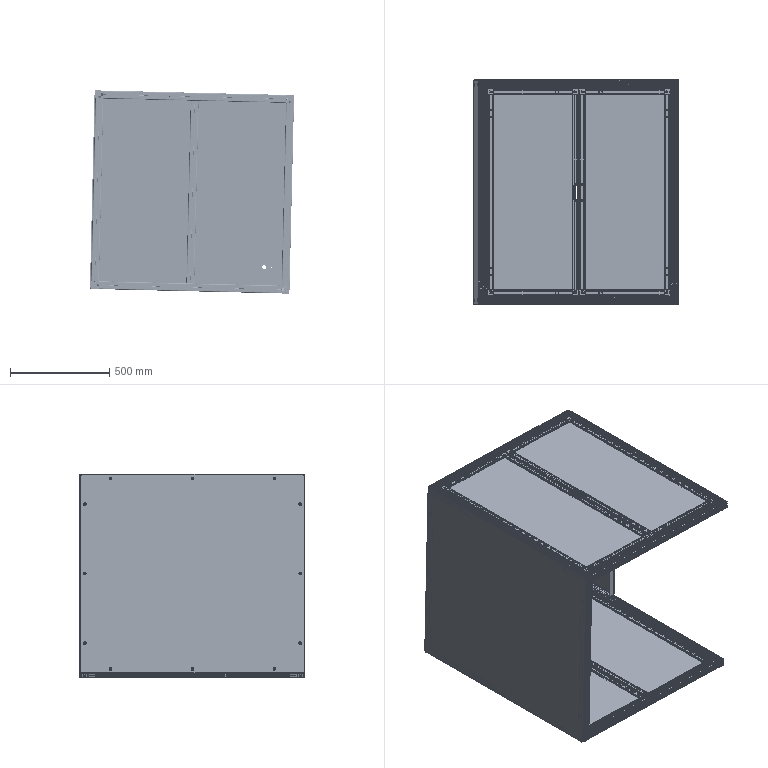Assembly | SolidWorks | mm | 149 component files | 149 solids | 6238 faces | box 1028.53 x 1130 x 1023.65 mm | volume 29494615 mm3 | plane 3910 | cylinder 1800 | cone 520 | spline 8 | commonest cylinder face diameters 6 x232 6.6 x230 2 x192 5 x184 11 x152 10 x120 6.8 x100 1 x96
Bill of materials:
1530ConnectorAMS12-1530 | 16 |  | Rectangular block with plain flat faces and round through-holes in its side faces.
ref18 | 4 | A6061 | Long, slender extruded bar with a rectangular cross-section and rounded corners. Each short side has an undercut slot pair, and there is a round bore through the center along its length. Small holes are grouped near both ends of one face.
AOB05-1530-L397 , Length 397mm | 2 | A6061 | Straight extruded bar with the same rounded-rectangle, two-slot cross-section and center bore as the slotted bars. No extra cutouts are visible along its length.
AOB05-1530-L397 , Length 397mm | 6 | A6061 | Straight extruded bar with a rounded-rectangle cross-section, undercut slots on two opposite sides and a central round bore. No extra cutouts are visible along its length.
1803ME3001 (Size:846*412*5mm) | 4 | PC | Thin flat rectangular plate with small step notches at each corner, so the short ends are slightly narrower.
AOB05-1530-L827-2 , Length 827mm | 4 | A6061 | Long extruded bar with the rounded-rectangle, two-slot cross-section and central bore. Mid-length, it has a rectangular cutout in one face with a small hole on each side of it.
HexSocketHeadCapScrewM6-16FerricOxide | 32 | SCM435 | Pin-shaped part with a short, larger-diameter cylindrical head and a smaller, longer cylindrical shank. Both ends are chamfered.
AOB05-4040-L920-LP-RP-LE-Z6-A70-B260-C260-D260 , Length 920mm | 1 | A6061 | Long extruded bar with a square cross-section, an undercut slot centered on each of the four sides, diagonal webs and a central bore with four radial notches. Small holes appear along one face and near the ends.
AOB05-4040-L920-LP-RP-LE-Z6-A70-B260-C260-D260 , Length 920mm | 2 | A6061 | Long extruded bar with a square cross-section, an undercut slot on each side, diagonal webs and a central notched bore. Small holes appear along one face and near the ends.
AOB05-4040-L970 , Length970mm | 4 | A6061 | Long straight extruded bar with a square cross-section, an undercut slot on each of the four sides, diagonal webs, hollow corner pockets and a central bore with four radial notches. No holes are visible along its length.
A3008 | 5 |  | Long straight extruded bar with a square cross-section, an undercut slot on each side, diagonal webs and a central notched bore. Small marks near the ends of one face may be holes.
Built-inConnectorADJ42-G408-D6.5 | 14 | S45C | Solid short cylinder with a round hole straight through its diameter. A thin rectangular tab sticks out sideways from the curved surface, flush with one end face.
HexSocketHeadCapScrewM6-25FerricOxide | 14 | SCM435 | Axisymmetric headed pin: short larger-diameter cylindrical head on a long, smooth, narrower cylindrical shank with a chamfered free end. Shaped like a cap-head screw blank.
RhombicNutAHG21-408-M6 | 14 |  | Rhombus/parallelogram-shaped block with one round through-hole near its center. The side profile is stepped, with a narrower raised tongue on one face. Two opposite corners of the outline are rounded and some edges are chamfered.
A3009 | 1 | PC | Thin, flat, nearly square plate with small rounded corners. It has a pattern of small holes spaced around the perimeter and one larger hole near a corner, surrounded by four small holes.
AHL21-308-M6 | 12 | S45C | Elongated half-round (D-section) body with a round through-hole crossing its curved side. A thin, angled flat flange extends from the top edge, and a small narrow rib or step runs along the flat back face. One edge has a semicircular notch where the hole breaks out.
HexSocketFlatHeadScrewM6-16FerrousOxide | 12 | SCM435 | Axisymmetric countersunk-head pin: a conical flat-topped head on a plain cylindrical shank with a chamfered tip. Shaped like a flat-head screw or rivet blank.
2403MA0512 | 1 | SUS304 | Tall rectangular bent-sheet panel with shallow depth, possibly a channel or tray shape with folded return flanges along its long sides. The main face has a rectangular cutout near the lower end, with a row of four round holes below it. The side flanges carry small round holes near the ends and the middle.
A3020 | 1 | PC | Thin, flat rectangular plate with small rounded corners and evenly spaced small holes around its perimeter, about three per edge. There are no interior features.
Mates:
1. coincident | assembly face at (597.759, -1214.138, 1384.919) dir (1, 0, 0) | assembly face at (597.759, -1307.138, 1248.419) dir (-1, 0, 0)
2. parallel | 2012MB0201-1/AUpperRackFrameModule-1/A3006-1 face at (-822.107, -81.15, -197.248) dir (0, -1, 0) | assembly plane at (0, 0, 0) dir (0, 1, 0)
3. coincident | 2012MB0201-1/AUpperRackFrameModule-1/A3007-2 face at (-1781.583, 1043.85, -163.887) dir (-0.9997, 0, 0.02392) | A3020-1 face at (-1793.436, 481.35, -659.245) dir (0.9997, 0, -0.02392)
4. coincident | 2012MB0201-1/AUpperRackFrameModule-1/A3007-2 face at (-1777.826, 1043.85, -194.986) dir (0, 1, 0) | A3020-1 face at (-1810.395, 1043.85, -1158.982) dir (0, 1, 0)
5. coincident | 2012MB0201-1/AUpperRackFrameModule-1/A3007-1 face at (-1800.898, 1043.85, -1159.21) dir (-0.02392, 0, -0.9997) | A3020-1 face at (-1810.395, 1043.85, -1158.982) dir (-0.02392, 0, -0.9997)
6. coincident | 2012MB0201-1/AUpperRackFrameModule-1/A3007-3 face at (-782.611, 1043.85, -218.799) dir (0.9997, 0, -0.02392) | 2403MA0512-1 face at (-793.722, 851.85, -683.166) dir (0.9997, 0, -0.02392)
7. coincident | 2012MB0201-1/AUpperRackFrameModule-1/A3008-3 face at (-787.217, 1003.85, -223.19) dir (0, -1, 0) | 2403MA0512-1 face at (-793.722, 1003.85, -683.166) dir (0, 1, 0)
8. distance | 2403MA0512-1 face at (-804.702, 851.85, -1142.035) dir (-0.02392, 0, -0.9997) | 2012MB0201-1/AUpperRackFrameModule-1/A3007-4 face at (-829.819, 1043.85, -1142.434) dir (0.02392, 0, 0.9997)
9. distance | ASideDoor-2-1/1530ConnectorAMS12-1530-8 face at (-482.615, 41.5, -1079.856) dir (0, -1, 0) | AUpperRackFrameModule-1/A3006-1 face at (-20.615, 40, -1084.356) dir (0, 1, 0)
10. distance | ASideDoor-2-1/1530ConnectorAMS12-1530-7 face at (-939.615, 41.5, -1094.856) dir (-1, 0, 0) | AUpperRackFrameModule-1/A3007-2 face at (-940.615, 1125, -1094.756) dir (1, 0, 0)
11. coincident | AUpperRackFrameModule-1/A3007-2 face at (-945.115, 1125, -1079.856) dir (0, 0, 1) | ASideDoor-2-1/A3001-4 face at (-939.615, 1053.5, -1079.856) dir (0, 0, 1)
12. distance | AUpperRackFrameModule-1/A3006-1 face at (-20.615, 40, -1084.356) dir (0, 1, 0) | ASideDoor-1-1/1530ConnectorAMS12-1530-8 face at (-21.615, 41.5, -1079.856) dir (0, -1, 0)
13. distance | ASideDoor-1-1/1530ConnectorAMS12-1530-8 face at (-21.615, 41.5, -1079.856) dir (1, 0, 0) | AUpperRackFrameModule-1/A3007-3 face at (-20.615, 1125, -1084.356) dir (-1, 0, 0)
14. coincident | AUpperRackFrameModule-1/A3007-3 face at (-5.715, 1125, -1079.856) dir (0, 0, 1) | ASideDoor-1-1/A3001-3 face at (-51.615, 1053.5, -1079.856) dir (0, 0, 1)
15. distance | UpperRackCoverModule-1/A3009-1 face at (-480.615, 1130, -1579.856) dir (0, 1, 0) | AUpperRackFrameModule-1/A3007-2 face at (-976.115, 1125, -1115.356) dir (0, 1, 0)
16. coincident | AUpperRackFrameModule-1/A3007-4 face at (-16.115, 1125, -2079.856) dir (0, 0, -1) | UpperRackCoverModule-1/A3009-1 face at (19.385, 1130, -2079.856) dir (0, 0, -1)
17. coincident | UpperRackCoverModule-1/A3009-1 face at (-980.615, 1130, -2079.856) dir (-1, 0, 0) | AUpperRackFrameModule-1/A3008-5 face at (-980.615, 1110.1, -1119.856) dir (-1, 0, 0)
18. parallel | AUpperRackFrameModule-1/A3008-6 face at (-20.615, 1120.5, -2063.956) dir (0, 0, 1) | UpperRackCoverModule-1/AHL21-308-M6-1 face at (-120.615, 1120.5, -2063.856) dir (0, 0, -1)
19. parallel | AUpperRackFrameModule-1/A3008-3 face at (3.485, 1120.5, -1119.856) dir (-1, 0, 0) | UpperRackCoverModule-1/AHL21-308-M6-2 face at (3.385, 1120.5, -1919.856) dir (1, 0, 0)
20. coincident | AUpperRackFrameModule-1/A3007-1 face at (-955.515, 1125, -2079.856) dir (0, 0, -1) | ASideDoor-1-3/A3001-3 face at (-909.115, 1053.5, -2079.856) dir (0, 0, -1)
21. coincident | ASideDoor-1-1/1530ConnectorAMS12-1530-5 face at (-478.615, 1083.5, -1079.856) dir (0, 1, 0) | ASideDoor-1-3/1530ConnectorAMS12-1530-5 face at (-482.115, 1083.5, -2079.856) dir (0, 1, 0)
22. coincident | AUpperRackFrameModule-1/A3007-4 face at (-16.115, 1125, -2079.856) dir (0, 0, -1) | ASideDoor-2-3/A3002-5 face at (-52.115, 1053.5, -2079.856) dir (0, 0, -1)
23. coincident | ASideDoor-2-3/1530ConnectorAMS12-1530-6 face at (-479.115, 1083.5, -2064.856) dir (0, 1, 0) | ASideDoor-1-3/1530ConnectorAMS12-1530-5 face at (-482.115, 1083.5, -2079.856) dir (0, 1, 0)
24. distance | ASideDoor-2-3/1530ConnectorAMS12-1530-5 face at (-22.115, 1083.5, -2079.856) dir (1, 0, 0) | AUpperRackFrameModule-1/A3007-4 face at (-20.615, 1125, -2064.956) dir (-1, 0, 0)
25. distance | ASideDoor-1-3/1530ConnectorAMS12-1530-6 face at (-939.115, 1083.5, -2064.856) dir (-1, 0, 0) | AUpperRackFrameModule-1/A3007-1 face at (-940.615, 1125, -2054.756) dir (1, 0, 0)
26. coincident | 2012MB0201 face at (-20.615, 0, -2075.356) dir (0, -1, 0) | 2012MB0201 plane at (0, 0, 0) dir (0, 1, 0)
27. coincident | A3005-1 face at (-200.853, 596.045, 717) dir (0, 1, 0) | 1530ConnectorAMS12-1530-5 face at (-215.853, 596.045, 724.5) dir (0, -1, 0)
28. coincident | A3005-1 face at (-215.853, 596.045, 724.5) dir (0, 0, 1) | 1530ConnectorAMS12-1530-5 face at (-200.853, 611.045, 724.5) dir (0, 0, 1)
29. coincident | A3005-1 face at (-215.853, 596.045, 709.5) dir (-1, 0, 0) | 1530ConnectorAMS12-1530-5 face at (-215.853, 626.045, 724.5) dir (-1, 0, 0)
30. coincident | A3001-3 face at (211.147, 596.045, 724.5) dir (0, 0, 1) | 1530ConnectorAMS12-1530-6 face at (226.147, 611.045, 724.5) dir (0, 0, 1)
31. coincident | A3001-3 face at (226.147, 596.045, 717) dir (0, 1, 0) | 1530ConnectorAMS12-1530-6 face at (241.147, 596.045, 709.5) dir (0, -1, 0)
32. coincident | A3001-3 face at (241.147, 596.045, 709.5) dir (1, 0, 0) | 1530ConnectorAMS12-1530-6 face at (241.147, 626.045, 709.5) dir (1, 0, 0)
33. coincident | A3005-1 face at (-200.853, -385.955, 717) dir (0, -1, 0) | 1530ConnectorAMS12-1530-7 face at (-215.853, -385.955, 709.5) dir (0, 1, 0)
34. coincident | A3001-3 face at (226.147, -385.955, 717) dir (0, -1, 0) | 1530ConnectorAMS12-1530-8 face at (241.147, -385.955, 724.5) dir (0, 1, 0)
35. distance | ASideDoor-1 face at (-61.253, -57.855, 719.5) dir (0, 0, 1) | A3005-1 face at (-185.853, 596.045, 720.25) dir (0, 0, -1)
36. distance | A3005-1 face at (-194.253, 596.045, 711.7) dir (1, 0, 0) | ASideDoor-1 face at (-194.253, 278.645, 719.5) dir (-1, 0, 0)
37. concentric | A3005-1 face at (-200.853, 69.545, 724.5) dir (0, 0, 1) r 2.5 | ASideDoor-1 face at (-200.853, 69.545, 724.5) dir (0, 0, 1) r 1.621
38. coincident | A3005-1 face at (-215.853, 596.045, 724.5) dir (0, 0, 1) | ASideDoor-1 face at (-196.353, 69.545, 724.5) dir (0, 0, -1)
39. parallel | 1530ConnectorAMS12-1530-8 face at (241.147, -415.955, 724.5) dir (0, -1, 0) | A3002-7 face at (211.147, -385.955, 709.5) dir (0, 1, 0)
40. coincident | A3005-1 face at (-215.853, 596.045, 709.5) dir (-1, 0, 0) | 1530ConnectorAMS12-1530-7 face at (-215.853, -415.955, 709.5) dir (-1, 0, 0)
41. coincident | A3001-3 face at (241.147, 596.045, 709.5) dir (1, 0, 0) | 1530ConnectorAMS12-1530-8 face at (241.147, -415.955, 724.5) dir (1, 0, 0)
42. coincident | A3005-1 face at (-215.853, 596.045, 709.5) dir (0, 0, -1) | 1530ConnectorAMS12-1530-7 face at (-200.853, -400.955, 709.5) dir (0, 0, -1)
43. coincident | A3005-1 face at (-215.853, 596.045, 724.5) dir (0, 0, 1) | A3002-7 face at (211.147, -385.955, 724.5) dir (0, 0, 1)
44. parallel | 1530ConnectorAMS12-1530-7 face at (-215.853, -415.955, 709.5) dir (0, -1, 0) | A3002-7 face at (211.147, -415.955, 709.5) dir (0, -1, 0)
45. coincident | A3005-1 face at (-185.853, 596.045, 709.5) dir (1, 0, 0) | A3002-7 face at (-185.853, -400.955, 717) dir (-1, 0, 0)
46. coincident | 1530ConnectorAMS12-1530-7 face at (-215.853, -415.955, 709.5) dir (0, -1, 0) | A3002-7 face at (211.147, -415.955, 709.5) dir (0, -1, 0)
47. coincident | A3001-3 face at (211.147, 596.045, 709.5) dir (0, 0, -1) | 1530ConnectorAMS12-1530-8 face at (226.147, -400.955, 709.5) dir (0, 0, -1)
48. coincident | 1530ConnectorAMS12-1530-6 face at (215.147, 611.045, 713.7) dir (1, 0, 0) | HexSocketHeadCapScrewM6-16FerricOxide-4 face at (215.147, 610.097, 712.091) dir (-1, 0, 0)
49. concentric | 1530ConnectorAMS12-1530-6 face at (226.147, 626.045, 717) dir (0, 1, 0) r 5.5 | HexSocketHeadCapScrewM6-16FerricOxide-3 face at (226.147, 600.045, 717) dir (0, 1, 0) r 5
50. coincident | 1530ConnectorAMS12-1530-6 face at (222.847, 600.045, 717) dir (0, 1, 0) | HexSocketHeadCapScrewM6-16FerricOxide-3 face at (226.867, 600.045, 712.052) dir (0, -1, 0)
51. coincident | 1530ConnectorAMS12-1530-5 face at (-189.853, 611.045, 720.3) dir (-1, 0, 0) | HexSocketHeadCapScrewM6-16FerricOxide-1 face at (-189.853, 613.137, 712.459) dir (1, 0, 0)
52. concentric | 1530ConnectorAMS12-1530-5 face at (-200.853, 626.045, 717) dir (0, 1, 0) r 5.5 | HexSocketHeadCapScrewM6-16FerricOxide-2 face at (-200.853, 500.045, 717) dir (0, 1, 0) r 3
53. coincident | 1530ConnectorAMS12-1530-5 face at (-197.553, 600.045, 717) dir (0, 1, 0) | HexSocketHeadCapScrewM6-16FerricOxide-2 face at (-205.814, 600.045, 716.38) dir (0, -1, 0)
54. concentric | 1530ConnectorAMS12-1530-7 face at (-200.853, -415.955, 717) dir (0, -1, 0) r 5.5 | HexSocketHeadCapScrewM6-16FerricOxide-5 face at (-200.853, -289.955, 717) dir (0, -1, 0) r 3
55. concentric | 1530ConnectorAMS12-1530-7 face at (-215.853, -400.955, 717) dir (-1, 0, 0) r 5.5 | HexSocketHeadCapScrewM6-16FerricOxide-6 face at (-89.853, -400.955, 717) dir (-1, 0, 0) r 3
56. coincident | 1530ConnectorAMS12-1530-7 face at (-189.853, -400.955, 713.7) dir (-1, 0, 0) | HexSocketHeadCapScrewM6-16FerricOxide-6 face at (-189.853, -400.955, 712) dir (1, 0, 0)
57. coincident | 1530ConnectorAMS12-1530-7 face at (-197.553, -389.955, 717) dir (0, -1, 0) | HexSocketHeadCapScrewM6-16FerricOxide-5 face at (-198.118, -389.955, 712.814) dir (0, 1, 0)
58. concentric | 1530ConnectorAMS12-1530-8 face at (241.147, -400.955, 717) dir (1, 0, 0) r 5.5 | HexSocketHeadCapScrewM6-16FerricOxide-7 face at (115.147, -400.955, 717) dir (1, 0, 0) r 3
59. coincident | 1530ConnectorAMS12-1530-8 face at (215.147, -400.955, 720.3) dir (1, 0, 0) | HexSocketHeadCapScrewM6-16FerricOxide-7 face at (215.147, -398.852, 712.464) dir (-1, 0, 0)
60. concentric | A3001-3 face at (226.147, 596.045, 717) dir (0, -1, 0) r 2.5 | HexSocketHeadCapScrewM6-16FerricOxide-8 face at (226.147, -289.955, 717) dir (0, -1, 0) r 3
61. coincident | 1530ConnectorAMS12-1530-8 face at (222.847, -389.955, 717) dir (0, -1, 0) | HexSocketHeadCapScrewM6-16FerricOxide-8 face at (229.723, -389.955, 720.495) dir (0, 1, 0)
62. coincident | 1530ConnectorAMS12-1530-5 face at (-185.853, 626.045, 724.5) dir (1, 0, 0) | A3002-0-1 face at (-185.853, 611.045, 717) dir (-1, 0, 0)
63. concentric | HexSocketHeadCapScrewM6-16FerricOxide-1 face at (-89.853, 611.045, 717) dir (-1, 0, 0) r 3 | A3002-0-1 face at (211.147, 611.045, 717) dir (-1, 0, 0) r 2.5
64. coincident | 1530ConnectorAMS12-1530-5 face at (-215.853, 626.045, 724.5) dir (0, 1, 0) | A3002-0-1 face at (211.147, 626.045, 709.5) dir (0, 1, 0)
65. coincident | 1530ConnectorAMS12-1530-6 face at (211.147, 626.045, 709.5) dir (-1, 0, 0) | A3002-0-1 face at (211.147, 611.045, 717) dir (1, 0, 0)
66. coincident | 1530ConnectorAMS12-1530-6 face at (241.147, 626.045, 709.5) dir (0, 1, 0) | A3002-0-1 face at (211.147, 626.045, 709.5) dir (0, 1, 0)
67. coincident | A3001-3 face at (211.147, 596.045, 724.5) dir (0, 0, 1) | A3002-0-1 face at (211.147, 626.045, 724.5) dir (0, 0, 1)
68. coincident | A3005-1 face at (-215.853, 596.045, 724.5) dir (0, 0, 1) | A3002-0-1 face at (211.147, 626.045, 724.5) dir (0, 0, 1)
69. coincident | A3001-4 face at (-200.853, 596.045, 717) dir (0, 1, 0) | 1530ConnectorAMS12-1530-5 face at (-215.853, 596.045, 724.5) dir (0, -1, 0)
70. coincident | A3001-4 face at (-215.853, 596.045, 724.5) dir (0, 0, 1) | 1530ConnectorAMS12-1530-5 face at (-200.853, 611.045, 724.5) dir (0, 0, 1)
71. coincident | A3001-4 face at (-215.853, 596.045, 709.5) dir (-1, 0, 0) | 1530ConnectorAMS12-1530-5 face at (-215.853, 626.045, 724.5) dir (-1, 0, 0)
72. coincident | A3002-5 face at (-185.853, 611.045, 717) dir (-1, 0, 0) | 1530ConnectorAMS12-1530-5 face at (-185.853, 626.045, 724.5) dir (1, 0, 0)
73. coincident | A3002-5 face at (-185.853, 596.045, 724.5) dir (0, 0, 1) | 1530ConnectorAMS12-1530-5 face at (-200.853, 611.045, 724.5) dir (0, 0, 1)
74. coincident | A3002-5 face at (-185.853, 626.045, 709.5) dir (0, 1, 0) | 1530ConnectorAMS12-1530-5 face at (-215.853, 626.045, 724.5) dir (0, 1, 0)
75. coincident | A3002-5 face at (211.147, 611.045, 717) dir (1, 0, 0) | 1530ConnectorAMS12-1530-6 face at (211.147, 626.045, 709.5) dir (-1, 0, 0)
76. coincident | A3002-5 face at (-185.853, 596.045, 724.5) dir (0, 0, 1) | 1530ConnectorAMS12-1530-6 face at (226.147, 611.045, 724.5) dir (0, 0, 1)
77. coincident | A3002-5 face at (-185.853, 626.045, 709.5) dir (0, 1, 0) | 1530ConnectorAMS12-1530-6 face at (241.147, 626.045, 709.5) dir (0, 1, 0)
78. coincident | A3005-2 face at (211.147, 596.045, 724.5) dir (0, 0, 1) | 1530ConnectorAMS12-1530-6 face at (226.147, 611.045, 724.5) dir (0, 0, 1)
79. coincident | A3005-2 face at (226.147, 596.045, 717) dir (0, 1, 0) | 1530ConnectorAMS12-1530-6 face at (241.147, 596.045, 709.5) dir (0, -1, 0)
80. coincident | A3005-2 face at (241.147, 596.045, 709.5) dir (1, 0, 0) | 1530ConnectorAMS12-1530-6 face at (241.147, 626.045, 709.5) dir (1, 0, 0)
81. coincident | A3001-4 face at (-215.853, 596.045, 724.5) dir (0, 0, 1) | A3002-6 face at (-185.853, -415.955, 724.5) dir (0, 0, 1)
82. coincident | A3001-4 face at (-185.853, 596.045, 709.5) dir (1, 0, 0) | A3002-6 face at (-185.853, -400.955, 717) dir (-1, 0, 0)
83. coincident | A3001-4 face at (-200.853, -385.955, 717) dir (0, -1, 0) | A3002-6 face at (-185.853, -385.955, 709.5) dir (0, 1, 0)
84. coincident | A3001-4 face at (-200.853, -385.955, 717) dir (0, -1, 0) | 1530ConnectorAMS12-1530-7 face at (-215.853, -385.955, 709.5) dir (0, 1, 0)
85. coincident | 1530ConnectorAMS12-1530-7 face at (-185.853, -415.955, 709.5) dir (1, 0, 0) | A3002-6 face at (-185.853, -400.955, 717) dir (-1, 0, 0)
86. coincident | 1530ConnectorAMS12-1530-7 face at (-200.853, -400.955, 724.5) dir (0, 0, 1) | A3002-6 face at (-185.853, -415.955, 724.5) dir (0, 0, 1)
87. coincident | A3005-2 face at (226.147, -385.955, 717) dir (0, -1, 0) | 1530ConnectorAMS12-1530-8 face at (241.147, -385.955, 724.5) dir (0, 1, 0)
88. coincident | 1530ConnectorAMS12-1530-8 face at (211.147, -415.955, 724.5) dir (-1, 0, 0) | A3002-6 face at (211.147, -400.955, 717) dir (1, 0, 0)
89. coincident | 1530ConnectorAMS12-1530-8 face at (226.147, -400.955, 724.5) dir (0, 0, 1) | A3002-6 face at (-185.853, -415.955, 724.5) dir (0, 0, 1)
90. width | A3002-6 face at (-185.853, -396.755, 714.074) dir (0, 1, 0) | A3002-5 face at (-185.853, 606.845, 714.074) dir (0, -1, 0) | A3004-2 face at (-193.353, -395.455, 719.5) dir (0, -1, 0) | A3004-2 face at (-193.353, 605.545, 719.5) dir (0, 1, 0)
91. width | A3001-4 face at (-196.653, 596.045, 714.074) dir (1, 0, 0) | A3005-2 face at (221.947, 596.045, 714.074) dir (-1, 0, 0) | A3004-2 face at (-193.353, 605.545, 719.5) dir (-1, 0, 0) | A3004-2 face at (218.647, 605.545, 719.5) dir (1, 0, 0)
92. width | A3005-2 face at (211.147, 596.045, 720.25) dir (0, 0, -1) | A3005-2 face at (211.147, 596.045, 713.75) dir (0, 0, 1) | A3004-2 face at (12.647, 105.045, 719.5) dir (0, 0, 1) | A3004-2 face at (12.647, 105.045, 714.5) dir (0, 0, -1)
93. concentric | 1530ConnectorAMS12-1530-8 face at (241.147, -400.955, 717) dir (1, 0, 0) r 5.5 | HexSocketHeadCapScrewM6-16FerricOxide-22 face at (215.147, -400.955, 717) dir (1, 0, 0) r 5
94. concentric | 1530ConnectorAMS12-1530-8 face at (226.147, -415.955, 717) dir (0, -1, 0) r 5.5 | HexSocketHeadCapScrewM6-16FerricOxide-23 face at (226.147, -389.955, 717) dir (0, -1, 0) r 5
95. coincident | 1530ConnectorAMS12-1530-8 face at (215.147, -400.955, 720.3) dir (1, 0, 0) | HexSocketHeadCapScrewM6-16FerricOxide-22 face at (215.147, -404.001, 720.965) dir (-1, 0, 0)
96. coincident | 1530ConnectorAMS12-1530-8 face at (222.847, -389.955, 717) dir (0, -1, 0) | HexSocketHeadCapScrewM6-16FerricOxide-23 face at (221.944, -389.955, 719.708) dir (0, 1, 0)
97. concentric | 1530ConnectorAMS12-1530-5 face at (-200.853, 626.045, 717) dir (0, 1, 0) r 5.5 | HexSocketHeadCapScrewM6-16FerricOxide-19 face at (-200.853, 500.045, 717) dir (0, 1, 0) r 3
98. coincident | 1530ConnectorAMS12-1530-5 face at (-197.553, 600.045, 717) dir (0, 1, 0) | HexSocketHeadCapScrewM6-16FerricOxide-19 face at (-204.91, 600.045, 719.922) dir (0, -1, 0)
99. concentric | 1530ConnectorAMS12-1530-7 face at (-215.853, -400.955, 717) dir (-1, 0, 0) r 5.5 | HexSocketHeadCapScrewM6-16FerricOxide-24 face at (-89.853, -400.955, 717) dir (-1, 0, 0) r 3
100. concentric | 1530ConnectorAMS12-1530-7 face at (-200.853, -415.955, 717) dir (0, -1, 0) r 5.5 | HexSocketHeadCapScrewM6-16FerricOxide-25 face at (-200.853, -289.955, 717) dir (0, -1, 0) r 3
101. coincident | 1530ConnectorAMS12-1530-7 face at (-197.553, -389.955, 717) dir (0, -1, 0) | HexSocketHeadCapScrewM6-16FerricOxide-25 face at (-205.36, -389.955, 719.164) dir (0, 1, 0)
102. coincident | 1530ConnectorAMS12-1530-7 face at (-189.853, -400.955, 713.7) dir (-1, 0, 0) | HexSocketHeadCapScrewM6-16FerricOxide-24 face at (-189.853, -398.844, 712.467) dir (1, 0, 0)
103. concentric | 1530ConnectorAMS12-1530-6 face at (241.147, 611.045, 717) dir (1, 0, 0) r 5.5 | HexSocketHeadCapScrewM6-16FerricOxide-21 face at (215.147, 611.045, 717) dir (1, 0, 0) r 5
104. coincident | 1530ConnectorAMS12-1530-6 face at (215.147, 611.045, 713.7) dir (1, 0, 0) | HexSocketHeadCapScrewM6-16FerricOxide-21 face at (215.147, 613.954, 721.067) dir (-1, 0, 0)
105. concentric | 1530ConnectorAMS12-1530-6 face at (226.147, 626.045, 717) dir (0, 1, 0) r 5.5 | HexSocketHeadCapScrewM6-16FerricOxide-20 face at (226.147, 600.045, 717) dir (0, 1, 0) r 5
106. coincident | 1530ConnectorAMS12-1530-6 face at (222.847, 600.045, 717) dir (0, 1, 0) | HexSocketHeadCapScrewM6-16FerricOxide-20 face at (231.141, 600.045, 716.755) dir (0, -1, 0)
107. concentric | 1530ConnectorAMS12-1530-5 face at (-215.853, 611.045, 717) dir (-1, 0, 0) r 5.5 | HexSocketHeadCapScrewM6-16FerricOxide-18 face at (-189.853, 611.045, 717) dir (-1, 0, 0) r 5
108. coincident | 1530ConnectorAMS12-1530-5 face at (-189.853, 611.045, 720.3) dir (-1, 0, 0) | HexSocketHeadCapScrewM6-16FerricOxide-18 face at (-189.853, 608.692, 721.412) dir (1, 0, 0)
109. coincident | A3006-1 face at (1026.374, 4.5, -29.823) dir (1, 0, 0) | A3007-2 face at (1026.374, 1125, -50.423) dir (-1, 0, 0)
110. coincident | A3006-1 face at (106.374, 25.1, -65.323) dir (0, 0, -1) | A3007-2 face at (1030.874, 1125, -65.323) dir (0, 0, -1)
111. coincident | A3006-1 face at (106.374, 4.5, -65.323) dir (0, 0, -1) | A3007-3 face at (91.474, 1125, -65.323) dir (0, 0, -1)
112. coincident | A3006-1 face at (106.374, 4.5, -29.823) dir (-1, 0, 0) | A3007-3 face at (106.374, 1125, -60.823) dir (1, 0, 0)
113. coincident | A3006-1 face at (106.374, 0, -50.423) dir (0, -1, 0) | A3007-2 face at (1061.874, 0, -29.823) dir (0, -1, 0)
114. coincident | A3006-1 face at (106.374, 4.5, -29.823) dir (-1, 0, 0) | A3007-3 face at (106.374, 1125, -60.823) dir (1, 0, 0)
115. coincident | A3006-1 face at (106.374, 0, -50.423) dir (0, -1, 0) | A3007-3 face at (101.874, 0, -29.823) dir (0, -1, 0)
116. coincident | A3006-1 face at (106.374, 40, -60.823) dir (0, 1, 0) | ADJ42-G408-D6.5Assembly-4/Built-inConnectorADJ42-G408-D6.5-1 face at (125.374, 40, -36.072) dir (0, 1, 0)
117. coincident | A3006-1 face at (106.374, 40, -40.223) dir (0, 1, 0) | ADJ42-G408-D6.5Assembly-5/Built-inConnectorADJ42-G408-D6.5-1 face at (1007.374, 40, -54.572) dir (0, 1, 0)
118. coincident | A3007-1 face at (1061.874, 1125, 934.677) dir (0, 0, 1) | A3008-6 face at (106.374, 1120.5, 934.677) dir (0, 0, 1)
119. coincident | A3007-1 face at (1026.374, 1125, 930.177) dir (-1, 0, 0) | A3008-6 face at (1026.374, 1089.5, 930.177) dir (1, 0, 0)
120. coincident | A3007-2 face at (1061.874, 1125, -29.823) dir (0, 1, 0) | A3008-5 face at (1041.274, 1125, -25.323) dir (0, 1, 0)
121. coincident | A3007-2 face at (1066.374, 1125, -60.823) dir (1, 0, 0) | A3008-5 face at (1066.374, 1110.1, -25.323) dir (1, 0, 0)
122. coincident | A3007-2 face at (1061.874, 1125, -25.323) dir (0, 0, 1) | A3008-5 face at (1030.874, 1089.5, -25.323) dir (0, 0, -1)
123. coincident | A3007-2 face at (1061.874, 1125, -29.823) dir (0, 1, 0) | A3008-7 face at (106.374, 1125, -40.223) dir (0, 1, 0)
124. coincident | A3007-2 face at (1051.474, 1125, -65.323) dir (0, 0, -1) | A3008-7 face at (106.374, 1110.1, -65.323) dir (0, 0, -1)
125. coincident | A3007-2 face at (1026.374, 1125, -50.423) dir (-1, 0, 0) | A3008-7 face at (1026.374, 1089.5, -29.823) dir (1, 0, 0)
126. coincident | A3007-2 face at (1030.874, 1125, -51.923) dir (1, 0, 0) | AUpperRackFrameModule face at (1031.124, 1125, -55.073) dir (-1, 0, 0)
127. width | AUpperRackFrameModule face at (1028.124, 1125, -41.323) dir (0, 0, 1) | AUpperRackFrameModule face at (1031.124, 1125, -49.323) dir (0, 0, -1) | A3007-2 face at (1030.874, 1125, -49.423) dir (0, 0, 1) | A3007-2 face at (1027.374, 1125, -41.223) dir (0, 0, -1)
128. coincident | A3007-2 edge at (1030.874, 1125, -41.223) dir (0, -1, 0) | AUpperRackFrameModule face at (1031.124, 42, -41.072) dir (-1, 0, 0)
129. coincident | A3007-2 face at (1061.874, 1125, -29.823) dir (0, 1, 0) | AUpperRackFrameModule face at (1037.624, 1125, -35.573) dir (0, 1, 0)
130. coincident | A3007-3 face at (101.874, 1125, -29.823) dir (0, 1, 0) | A3008-3 face at (101.874, 1125, -25.323) dir (0, 1, 0)
131. coincident | A3007-3 face at (66.374, 1125, -50.423) dir (-1, 0, 0) | A3008-3 face at (66.374, 1120.5, -25.323) dir (-1, 0, 0)
132. coincident | A3007-3 face at (101.874, 1125, -25.323) dir (0, 0, 1) | A3008-3 face at (70.874, 1089.5, -25.323) dir (0, 0, -1)
133. coincident | A3007-3 face at (101.874, 1125, -49.423) dir (-1, 0, 0) | AUpperRackFrameModule face at (102.124, 1125, -49.572) dir (1, 0, 0)
134. width | A3007-3 face at (90.474, 1125, -26.323) dir (-1, 0, 0) | A3007-3 face at (82.274, 1125, -29.823) dir (1, 0, 0) | AUpperRackFrameModule face at (82.624, 1125, -29.823) dir (-1, 0, 0) | AUpperRackFrameModule face at (90.624, 1125, -26.823) dir (1, 0, 0)
135. coincident | A3007-3 face at (90.474, 1125, -29.823) dir (0, 0, -1) | AUpperRackFrameModule face at (90.624, 1125, -29.823) dir (0, 0, 1)
136. coincident | A3007-3 face at (101.874, 1125, -29.823) dir (0, 1, 0) | AUpperRackFrameModule face at (95.624, 1125, -55.322) dir (0, 1, 0)
137. coincident | A3007-3 edge at (101.874, 1125, -41.223) dir (0, -1, 0) | AUpperRackFrameModule face at (106.729, 42, -28.427) dir (0.9409, 0, -0.3386)
138. coincident | A3007-3 face at (101.874, 1125, -29.823) dir (0, 1, 0) | AUpperRackFrameModule face at (96.374, 1125, -36.323) dir (0, 1, 0)
139. coincident | A3007-4 face at (101.874, 1125, 930.177) dir (0, 1, 0) | A3008-6 face at (106.374, 1125, 899.177) dir (0, 1, 0)
140. coincident | A3007-4 face at (70.874, 1125, 894.677) dir (0, 0, -1) | A3008-3 face at (70.874, 1089.5, 894.677) dir (0, 0, 1)
141. coincident | A3007-4 face at (106.374, 1125, 919.777) dir (1, 0, 0) | A3008-6 face at (106.374, 1089.5, 930.177) dir (-1, 0, 0)
142. coincident | A3007-4 face at (101.874, 1125, 934.677) dir (0, 0, 1) | A3008-6 face at (106.374, 1120.5, 934.677) dir (0, 0, 1)
143. width | A3007-4 face at (82.274, 1125, 895.677) dir (1, 0, 0) | A3007-4 face at (90.474, 1125, 899.177) dir (-1, 0, 0) | AUpperRackFrameModule face at (82.374, 1125, 896.177) dir (-1, 0, 0) | AUpperRackFrameModule face at (90.374, 1125, 899.177) dir (1, 0, 0)
144. coincident | A3007-4 face at (82.274, 1125, 899.177) dir (0, 0, 1) | AUpperRackFrameModule face at (82.374, 1125, 899.177) dir (0, 0, -1)
145. coincident | A3007-4 face at (101.874, 1125, 930.177) dir (0, 1, 0) | AUpperRackFrameModule face at (76.624, 1125, 905.677) dir (0, 1, 0)
146. concentric | A3008-7 face at (125.374, 1107, -45.322) dir (0, 1, 0) r 9.5 | ADJ42-G408-D6.5Assembly-1/Built-inConnectorADJ42-G408-D6.5-1 face at (125.374, 1123, -45.322) dir (0, -1, 0) r 9.25
147. coincident | A3008-7 face at (106.374, 1125, -40.223) dir (0, 1, 0) | A3008-8 face at (581.874, 1125, -25.323) dir (0, 1, 0)
148. coincident | A3008-7 face at (106.374, 1120.5, -25.323) dir (0, 0, 1) | A3008-8 face at (550.874, 1120.5, -25.323) dir (0, 0, -1)
149. concentric | A3008-5 face at (1046.373, 1107, -6.323) dir (0, 1, 0) r 9.5 | ADJ42-G408-D6.5Assembly-12/Built-inConnectorADJ42-G408-D6.5-1 face at (1046.373, 1123, -6.323) dir (0, -1, 0) r 9.25
150. concentric | A3008-6 face at (1007.374, 1107, 914.678) dir (0, 1, 0) r 9.5 | ADJ42-G408-D6.5Assembly-10/Built-inConnectorADJ42-G408-D6.5-1 face at (1007.374, 1123, 914.678) dir (0, -1, 0) r 9.25
151. concentric | A3008-5 face at (1046.373, 1107, 875.677) dir (0, 1, 0) r 9.5 | ADJ42-G408-D6.5Assembly-11/Built-inConnectorADJ42-G408-D6.5-1 face at (1046.373, 1123, 875.677) dir (0, -1, 0) r 9.25
152. coincident | AUpperRackFrameModule face at (1056.624, 1125, -36.323) dir (0, 1, 0) | A3008-5 face at (1041.274, 1125, -25.323) dir (0, 1, 0)
153. coincident | A3008-6 face at (106.374, 1125, 899.177) dir (0, 1, 0) | AUpperRackFrameModule face at (1037.374, 1125, 924.678) dir (0, 1, 0)
154. coincident | A3008-6 face at (106.374, 1125, 899.177) dir (0, 1, 0) | AUpperRackFrameModule face at (95.374, 1125, 904.678) dir (0, 1, 0)
155. concentric | A3008-6 face at (125.374, 1107, 914.678) dir (0, 1, 0) r 9.5 | ADJ42-G408-D6.5Assembly-9/Built-inConnectorADJ42-G408-D6.5-1 face at (125.374, 1123, 914.678) dir (0, -1, 0) r 9.25
156. concentric | A3008-8 face at (568.374, 1105.001, 875.677) dir (1, 0, 0) r 9.5 | ADJ42-G408-D6.5Assembly-14/Built-inConnectorADJ42-G408-D6.5-1 face at (584.624, 1105.001, 875.677) dir (-1, 0, 0) r 9.25
157. coincident | A3008-8 face at (586.374, 1089.5, -25.323) dir (1, 0, 0) | AUpperRackFrameModule face at (586.624, 1115.001, 905.677) dir (1, 0, 0)
158. parallel | A3008-8 face at (550.874, 1120.5, 894.677) dir (0, 0, 1) | AUpperRackFrameModule face at (586.624, 1095.501, 899.177) dir (0, 0, -1)
159. concentric | A3008-8 face at (568.374, 1105.001, -6.323) dir (1, 0, 0) r 9.5 | ADJ42-G408-D6.5Assembly-13/Built-inConnectorADJ42-G408-D6.5-1 face at (584.624, 1105.001, -6.323) dir (-1, 0, 0) r 9.25
160. coincident | A3008-8 face at (586.374, 1089.5, -25.323) dir (1, 0, 0) | AUpperRackFrameModule face at (586.624, 1095.001, -36.323) dir (1, 0, 0)
161. parallel | A3008-8 face at (585.374, 1100.9, -25.323) dir (0, 1, 0) | AUpperRackFrameModule face at (586.624, 1108.751, -29.823) dir (0, 1, 0)
162. concentric | A3006-1 face at (125.374, 22, -45.322) dir (0, 1, 0) r 9.5 | ADJ42-G408-D6.5Assembly-4/Built-inConnectorADJ42-G408-D6.5-1 face at (125.374, 40, -45.322) dir (0, -1, 0) r 9.25
163. coincident | A3007-4 edge at (101.874, 1125, 918.777) dir (0, -1, 0) | AUpperRackFrameModule face at (101.874, 42, 910.677) dir (1, 0, 0)
164. width | A3008-8 face at (546.374, 1120.5, -25.323) dir (-1, 0, 0) | A3008-8 face at (586.374, 1110.1, -25.323) dir (1, 0, 0) | A3008-3 face at (106.374, 1110.1, -25.323) dir (1, 0, 0) | A3008-5 face at (1026.374, 1120.5, -25.323) dir (-1, 0, 0)
165. coincident | A3007-1 face at (1061.874, 1125, 930.177) dir (0, 1, 0) | A3008-5 face at (1061.874, 1125, -25.323) dir (0, 1, 0)
166. concentric | A3006-1 face at (1007.374, 22, -45.322) dir (0, 1, 0) r 9.5 | ADJ42-G408-D6.5Assembly-5/Built-inConnectorADJ42-G408-D6.5-1 face at (1007.374, 40, -45.322) dir (0, -1, 0) r 9.25
167. parallel | A3007-3 face at (66.374, 1125, -50.423) dir (-1, 0, 0) | AUpperRackFrameModule plane at (0, 0, 0) dir (1, 0, 0)
168. coincident | A3007-4 face at (106.374, 1125, 919.777) dir (1, 0, 0) | A3006-0-1 face at (106.374, 4.5, 930.177) dir (-1, 0, 0)
169. coincident | A3007-4 face at (101.874, 1125, 934.677) dir (0, 0, 1) | A3006-0-1 face at (106.374, 35.5, 934.677) dir (0, 0, 1)
170. parallel | A3007-3 face at (101.874, 1125, -41.223) dir (0, 0, -1) | ADJ42-G408-D6.5Assembly-4/Built-inConnectorADJ42-G408-D6.5-1 face at (134.626, 40, -49.322) dir (0, 0, -1)
171. coincident | A3006-0-1 face at (106.374, 40, 919.777) dir (0, 1, 0) | A3006-5 face at (1051.474, 40, 894.677) dir (0, 1, 0)
172. coincident | A3007-1 face at (1066.374, 1125, 899.177) dir (1, 0, 0) | A3006-5 face at (1066.374, 35.5, 894.677) dir (1, 0, 0)
173. coincident | A3007-1 face at (1051.474, 1125, 894.677) dir (0, 0, -1) | A3006-5 face at (1061.874, 4.5, 894.677) dir (0, 0, 1)
174. coincident | A3007-1 face at (1066.374, 1125, 899.177) dir (1, 0, 0) | A3006-5 face at (1066.374, 35.5, 894.677) dir (1, 0, 0)
175. coincident | A3007-1 face at (1066.374, 1125, 899.177) dir (1, 0, 0) | A3008-5 face at (1066.374, 1110.1, -25.323) dir (1, 0, 0)
176. coincident | A3008-5 face at (1046.373, 1107, 875.677) dir (0, 1, 0) | ADJ42-G408-D6.5Assembly-11/Built-inConnectorADJ42-G408-D6.5-1 face at (1046.373, 1107, 875.677) dir (0, -1, 0)
177. concentric | Built-inConnectorADJ42-G408-D6.5-1 face at (529.509, -1420.138, 687.919) dir (-1, 0, 0) r 3.25 | HexSocketHeadCapScrewM6-25FerricOxide-1 face at (641.509, -1420.138, 687.919) dir (-1, 0, 0) r 3
178. coincident | Built-inConnectorADJ42-G408-D6.5-1 face at (541.509, -1416.888, 687.919) dir (-1, 0, 0) | HexSocketHeadCapScrewM6-25FerricOxide-1 face at (541.509, -1418.229, 683.298) dir (1, 0, 0)
179. parallel | Built-inConnectorADJ42-G408-D6.5-1 face at (529.507, -1426.138, 691.919) dir (0, 0, 1) | RhombicNutAHG21-408-M6-1 face at (562.259, -1418.141, 694.669) dir (0, 0, 1)
180. distance | RhombicNutAHG21-408-M6-1 face at (562.259, -1418.141, 690.669) dir (-1, 0, 0) | Built-inConnectorADJ42-G408-D6.5-1 face at (557.259, -1428.138, 687.919) dir (1, 0, 0)
181. concentric | HexSocketHeadCapScrewM6-25FerricOxide-1 face at (641.509, -1420.138, 687.919) dir (-1, 0, 0) r 3 | RhombicNutAHG21-408-M6-1 face at (568.259, -1420.138, 687.919) dir (-1, 0, 0) r 3
182. coincident | A3009-1 face at (635.46, -1435.988, 1482.765) dir (0, 1, 0) r 785.398 | HexSocketFlatHeadScrewM6-16FerrousOxide-1 face at (635.46, -1435.688, 1482.765) dir (0, 1, 0) r 785.398
183. coincident | A3009-1 face at (505.46, -1435.988, 1612.765) dir (0, 1, 0) r 785.398 | HexSocketFlatHeadScrewM6-16FerrousOxide-13 face at (505.46, -1435.688, 1612.765) dir (0, 1, 0) r 785.398
184. concentric | AHL21-308-M6-1 face at (505.46, -1420.988, 1612.765) dir (0, 1, 0) r 3 | HexSocketFlatHeadScrewM6-16FerrousOxide-13 face at (505.46, -1395.988, 1612.765) dir (0, -1, 0) r 3
185. distance | AHL21-308-M6-1 face at (515.46, -1426.488, 1606.786) dir (0, -1, 0) | A3009-1 face at (155.46, -1430.988, 1132.765) dir (0, 1, 0)
186. concentric | HexSocketFlatHeadScrewM6-16FerrousOxide-1 face at (635.46, -1395.988, 1482.765) dir (0, -1, 0) r 3 | AHL21-308-M6-2 face at (635.46, -1420.988, 1482.765) dir (0, 1, 0) r 3
187. coincident | AHL21-308-M6-1 face at (515.46, -1426.988, 1608.765) dir (0, -1, 0) | AHL21-308-M6-2 face at (631.461, -1426.988, 1472.765) dir (0, -1, 0)